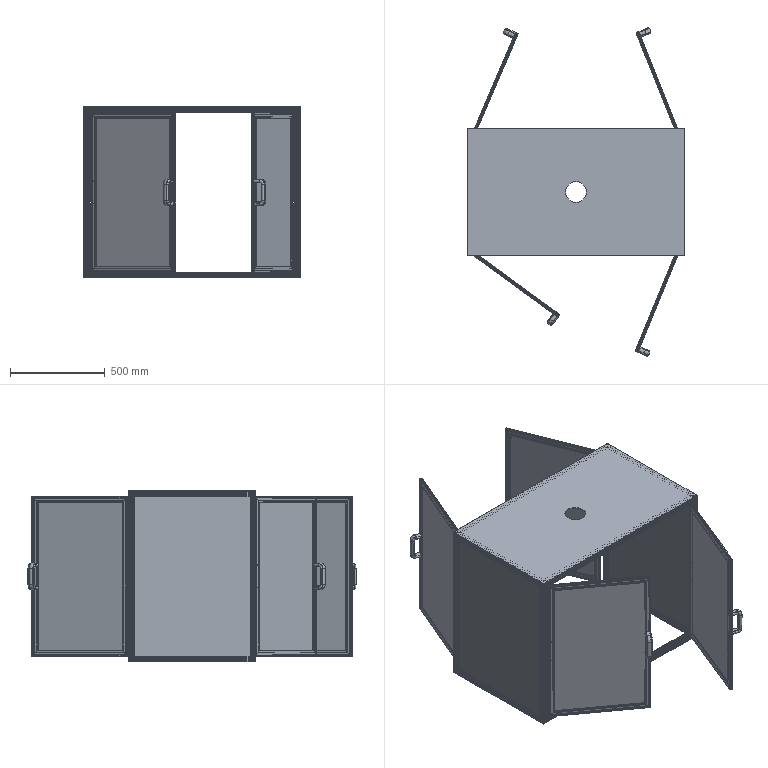Assembly | SolidWorks | mm | 39 component files | 39 solids | 1600 faces | box 1145 x 1728.9 x 905 mm | volume 23832016 mm3 | plane 1146 | cylinder 358 | cone 64 | spline 32 | commonest cylinder face diameters 4.2 x96 0.6 x48 4 x48 5 x32 1 x32 6.8 x24 42 x24 15.54 x20
Bill of materials:
3030-1085 | 4 |  | Long straight prismatic bar with a constant square cross-section: a central round bore, four round corner bores, diagonal webs, and an open slot centered on each of the four faces.
3030-610 | 4 |  | Straight prismatic bar with the same square, four-slot cross-section (central bore, four corner bores, diagonal webs). It looks shorter relative to its section than unnamed part.
3030-900 | 4 |  | Long straight bar with the same square, four-slot cross-section (central bore, four corner bores, diagonal webs), shown standing vertically.
858X628X5 | 2 |  | Thin, flat rectangular plate or sheet with no visible holes or cutouts.
3015-542.5 | 8 |  | Long, narrow slotted strip or profile. Both ends are cut at an angle, giving a trapezoid outline in side view, and grooves run along its length.
3015-840 | 8 |  | Long, slender extrusion with an elongated rectangular cross-section: one central round hole and open lipped slots at both ends and along the sides. The section view appears tilted.
503.5-801-5 | 4 |  | Thin, flat rectangular plate with no visible holes or cutouts.
TopCoverPlate | 1 |  | Thin, flat rectangular plate with one centered circular through-hole.
UPCFN120Handle | 4 |  | U-shaped (bow) handle made of a round-section bar: two parallel legs joined by a straight grip section with rounded bends. Each leg end has a small axial hole.
Mates:
1. coincident | 3030-900-1 face at (1.276, -17.477, 450) dir (0, -1, 0) | 3030-900-2 face at (1097.953, -17.477, 450) dir (0, -1, 0)
2. coincident | 3030-900-1 face at (-27.747, 1.323, 450) dir (0, 0, 1) | 3030-900-2 face at (1087.253, 1.323, 450) dir (0, 0, 1)
3. coincident | 3030-900-1 face at (-27.747, 1.323, 450) dir (0, 0, 1) | 3030-900-4 face at (-27.747, 641.323, 450) dir (0, 0, 1)
4. coincident | 3030-900-1 face at (-28.047, -15.977, 450) dir (-1, 0, 0) | 3030-900-4 face at (-28.047, 641.323, 450) dir (-1, 0, 0)
5. coincident | 3030-900-2 face at (1087.253, 1.323, 450) dir (0, 0, 1) | 3030-900-3 face at (1087.253, 641.323, 450) dir (0, 0, 1)
6. coincident | 3030-900-2 face at (1116.953, -7.277, 450) dir (1, 0, 0) | 3030-900-3 face at (1116.953, 651.023, 450) dir (1, 0, 0)
7. coincident | 3030-900-3 face at (1087.631, 652.523, 450) dir (0, 1, 0) | 3030-900-4 face at (-9.047, 652.523, 450) dir (0, 1, 0)
8. coincident | 3030-900-1 face at (1.953, -7.277, 450) dir (1, 0, 0) | 3030-1085-1 face at (1.953, 1.323, -449.7) dir (-1, 0, 0)
9. coincident | 3030-900-1 face at (1.276, -17.477, 450) dir (0, -1, 0) | 3030-1085-1 face at (1.953, -17.477, -439) dir (0, -1, 0)
10. coincident | 3030-900-1 face at (-27.747, 1.323, -450) dir (0, 0, -1) | 3030-1085-1 face at (1.953, -15.977, -450) dir (0, 0, -1)
11. coincident | 3030-900-2 face at (1086.953, 1.323, 450) dir (-1, 0, 0) | 3030-1085-1 face at (1086.953, 1.323, -449.7) dir (1, 0, 0)
12. coincident | 3030-900-4 face at (1.953, 632.723, 450) dir (1, 0, 0) | 3030-1085-2 face at (1.953, 641.323, -449.7) dir (-1, 0, 0)
13. coincident | 3030-900-4 face at (1.276, 622.523, 450) dir (0, -1, 0) | 3030-1085-2 face at (1.953, 622.523, -439) dir (0, -1, 0)
14. coincident | 3030-900-4 face at (-27.747, 641.323, -450) dir (0, 0, -1) | 3030-1085-2 face at (1.953, 624.023, -450) dir (0, 0, -1)
15. coincident | 3030-900-1 face at (1.953, 11.023, 450) dir (1, 0, 0) | 3030-1085-3 face at (1.953, 1.323, 420.3) dir (-1, 0, 0)
16. coincident | 3030-900-1 face at (1.276, -17.477, 450) dir (0, -1, 0) | 3030-1085-3 face at (1.953, -17.477, 449.323) dir (0, -1, 0)
17. coincident | 3030-900-1 face at (-27.747, 1.323, 450) dir (0, 0, 1) | 3030-1085-3 face at (1.953, 11.023, 450) dir (0, 0, 1)
18. coincident | 3030-900-4 face at (1.953, 632.723, 450) dir (1, 0, 0) | 3030-1085-5 face at (1.953, 641.323, 420.3) dir (-1, 0, 0)
19. coincident | 3030-900-4 face at (1.276, 622.523, 450) dir (0, -1, 0) | 3030-1085-5 face at (1.953, 622.523, 449.323) dir (0, -1, 0)
20. coincident | 3030-900-4 face at (-27.747, 641.323, 450) dir (0, 0, 1) | 3030-1085-5 face at (1.953, 651.023, 450) dir (0, 0, 1)
21. coincident | 3030-1085-2 face at (1.953, 622.523, -439) dir (0, -1, 0) | 3030-610-1 face at (-27.747, 622.523, -438.8) dir (0, 1, 0)
22. coincident | 3030-900-4 face at (-28.047, 624.023, 450) dir (-1, 0, 0) | 3030-610-1 face at (-28.047, 622.523, -438.8) dir (-1, 0, 0)
23. coincident | 3030-900-4 face at (-27.747, 641.323, -450) dir (0, 0, -1) | 3030-610-1 face at (-9.047, 622.523, -450) dir (0, 0, -1)
24. coincident | 3030-900-1 face at (-9.047, 12.523, 450) dir (0, 1, 0) | 3030-610-1 face at (-27.747, 12.523, -438.8) dir (0, -1, 0)
25. coincident | 3030-900-2 face at (1105.953, 12.523, 450) dir (0, 1, 0) | 3030-610-4 face at (1087.253, 12.523, -431.2) dir (0, -1, 0)
26. coincident | 3030-900-2 face at (1116.953, 11.023, 450) dir (1, 0, 0) | 3030-610-4 face at (1116.953, 12.523, -439.8) dir (1, 0, 0)
27. coincident | 3030-900-2 face at (1087.253, 1.323, -450) dir (0, 0, -1) | 3030-610-4 face at (1116.276, 12.523, -450) dir (0, 0, -1)
28. coincident | 3030-900-3 face at (1116.276, 622.523, 450) dir (0, -1, 0) | 3030-610-3 face at (1087.253, 622.523, 431.2) dir (0, 1, 0)
29. coincident | 3030-900-3 face at (1116.953, 651.023, 450) dir (1, 0, 0) | 3030-610-3 face at (1116.953, 622.523, 421.5) dir (1, 0, 0)
30. coincident | 3030-900-3 face at (1087.253, 641.323, 450) dir (0, 0, 1) | 3030-610-3 face at (1097.953, 622.523, 450) dir (0, 0, 1)
31. coincident | 3030-900-4 face at (-17.047, 622.523, 450) dir (0, -1, 0) | 3030-610-2 face at (-27.747, 622.523, 431.2) dir (0, 1, 0)
32. coincident | 3030-900-4 face at (-28.047, 624.023, 450) dir (-1, 0, 0) | 3030-610-2 face at (-28.047, 622.523, 431.2) dir (-1, 0, 0)
33. coincident | 3030-900-4 face at (-27.747, 641.323, 450) dir (0, 0, 1) | 3030-610-2 face at (1.276, 622.523, 450) dir (0, 0, 1)
34. coincident | 3030-610-3 face at (1097.953, 622.523, 450) dir (0, 0, 1) | TopCoverPlate-1 face at (-28.047, 652.523, 450) dir (0, 0, -1)
35. coincident | 3030-610-3 face at (1116.953, 622.523, 439.8) dir (1, 0, 0) | TopCoverPlate-1 face at (1116.953, 652.523, 455) dir (1, 0, 0)
36. coincident | 3030-900-3 face at (1105.953, 652.523, 450) dir (0, 1, 0) | TopCoverPlate-1 face at (-28.047, 652.523, 455) dir (0, 1, 0)
37. coincident | 3030-610-4 face at (1097.368, 12.523, -429) dir (0, 0, 1) | 858X628X5-1 face at (1105.953, 631.523, -429) dir (0, 0, -1)
38. coincident | 3030-900-3 face at (1106.539, 631.523, 450) dir (0, -1, 0) | 858X628X5-1 face at (1105.953, 631.523, 429) dir (0, 1, 0)
39. coincident | 3030-610-4 face at (1105.953, 12.523, -422) dir (-1, 0, 0) | 858X628X5-1 face at (1105.953, 631.523, 429) dir (1, 0, 0)
40. coincident | 3030-610-1 face at (-8.461, 622.523, -429) dir (0, 0, 1) | 858X628X5-2 face at (-17.047, 631.523, -429) dir (0, 0, -1)
41. coincident | 3030-900-1 face at (-17.632, 3.523, 450) dir (0, 1, 0) | 858X628X5-2 face at (-17.047, 3.523, -429) dir (0, -1, 0)
42. coincident | 3030-610-1 face at (-17.047, 622.523, -422) dir (1, 0, 0) | 858X628X5-2 face at (-17.047, 631.523, -429) dir (-1, 0, 0)
43. coincident | 3030-1085-5 face at (1.953, 624.023, 420) dir (0, 0, -1) | GuardDoor-1/3015-542.5-1 face at (1067.141, 655.276, 420) dir (0, 0, 1)
44. coincident | 3030-1085-5 face at (1.953, 624.023, 420) dir (0, 0, -1) | GuardDoor-2/3015-542.5-1 face at (235.292, 1153.537, 420) dir (0, 0, 1)
45. coincident | GuardDoor-1/3015-840-1 face at (875.161, 1162.783, -420) dir (0.9282, 0.3721, 0) | UPCFN120Handle-1 face at (880.742, 1148.86, -60.5) dir (-0.9282, -0.3721, 0)
46. concentric | GuardDoor-1/3015-840-1 face at (867.283, 1143.465, 60) dir (-0.9282, -0.3721, 0) r 0.5 | UPCFN120Handle-1 face at (891.874, 1153.323, 60) dir (-0.9282, -0.3721, 0) r 3.324
47. concentric | GuardDoor-1/3015-840-1 face at (867.283, 1143.465, -60) dir (-0.9282, -0.3721, 0) r 0.5 | UPCFN120Handle-1 face at (891.874, 1153.323, -60) dir (-0.9282, -0.3721, 0) r 3.324
48. coincident | GuardDoor-2/3015-840-2 face at (225.502, 1157.731, -420) dir (-0.9192, 0.3938, 0) | UPCFN120Handle-2 face at (219.596, 1143.943, -60.5) dir (0.9192, -0.3938, 0)
49. concentric | GuardDoor-2/3015-840-2 face at (220.055, 1143.746, -60) dir (-0.9192, 0.3938, 0) r 0.5 | UPCFN120Handle-2 face at (208.572, 1148.666, -60) dir (0.9192, -0.3938, 0) r 3.324
50. concentric | GuardDoor-2/3015-840-2 face at (220.055, 1143.746, 60) dir (-0.9192, 0.3938, 0) r 0.5 | UPCFN120Handle-2 face at (208.572, 1148.666, 60) dir (0.9192, -0.3938, 0) r 3.324
51. coincident | 3030-1085-3 face at (1.953, 1.323, 420) dir (0, 0, -1) | GuardDoor-4/3015-542.5-1 face at (457.672, -327.96, 420) dir (0, 0, 1)
52. coincident | 3030-1085-3 face at (1.953, -15.977, 420) dir (0, 0, -1) | GuardDoor-3/3015-542.5-1 face at (1063.157, -18.418, 420) dir (0, 0, 1)
53. coincident | GuardDoor-3/3015-840-1 face at (870.61, -525.82, -420) dir (0.9248, -0.3805, 0) | UPCFN120Handle-3 face at (876.318, -511.948, -60.5) dir (-0.9248, 0.3805, 0)
54. concentric | GuardDoor-3/3015-840-1 face at (875.855, -511.758, 60) dir (0.9248, -0.3805, 0) r 0.5 | UPCFN120Handle-3 face at (887.409, -516.512, 60) dir (-0.9248, 0.3805, 0) r 3.324
55. concentric | GuardDoor-3/3015-840-1 face at (875.855, -511.758, -60) dir (0.9248, -0.3805, 0) r 0.5 | UPCFN120Handle-3 face at (887.409, -516.512, -60) dir (-0.9248, 0.3805, 0) r 3.324
56. coincident | GuardDoor-4/3015-840-2 face at (448.83, -340.077, -420) dir (-0.5895, -0.8078, 0) | UPCFN120Handle-4 face at (436.713, -331.236, 60.5) dir (0.5895, 0.8078, 0)
57. concentric | GuardDoor-4/3015-840-2 face at (445.26, -319.522, 60) dir (0.5895, 0.8078, 0) r 0.5 | UPCFN120Handle-4 face at (429.643, -340.923, 60) dir (0.5895, 0.8078, 0) r 3.324
58. concentric | GuardDoor-4/3015-840-2 face at (445.26, -319.522, -60) dir (0.5895, 0.8078, 0) r 0.5 | UPCFN120Handle-4 face at (429.643, -340.923, -60) dir (0.5895, 0.8078, 0) r 3.324
59. coincident | 3030-1085-5 face at (1.953, 624.023, 420) dir (0, 0, -1) | GuardDoor-1/3015-542.5-1 face at (1077.026, 659.239, 420) dir (0, 0, 1)
60. coincident | 3015-542.5-1 face at (-16.364, -10.026, -271.25) dir (0.7071, 0, -0.7071) | 3015-840-1 face at (13.636, 29.974, -241.25) dir (-0.7071, 0, 0.7071)
61. coincident | 3015-542.5-1 face at (-16.364, 7.974, 271.25) dir (0, 1, 0) | 3015-840-1 face at (823.636, 7.974, -271.25) dir (0, 1, 0)
62. coincident | 3015-542.5-1 face at (-16.364, 7.974, 271.25) dir (-1, 0, 0) | 3015-840-1 edge at (-16.364, 3.624, -271.25) dir (0, 1, 0)
63. coincident | 3015-542.5-1 face at (-16.364, 7.974, 271.25) dir (0, 1, 0) | 3015-840-2 face at (823.636, 7.974, 271.25) dir (0, 1, 0)
64. coincident | 3015-542.5-1 face at (-16.364, -10.026, 271.25) dir (0.7071, 0, 0.7071) | 3015-840-2 face at (13.636, -29.026, 241.25) dir (-0.7071, 0, -0.7071)
65. coincident | 3015-542.5-1 face at (-16.364, 7.974, 271.25) dir (-1, 0, 0) | 3015-840-2 edge at (-16.364, 7.974, 271.25) dir (0, -1, 0)
66. coincident | 3015-840-2 face at (823.636, -7.026, 271.25) dir (0, -1, 0) | 3015-542.5-2 face at (823.636, -7.026, 271.25) dir (0, -1, 0)
67. coincident | 3015-840-2 face at (823.636, -13.026, 271.25) dir (0.7071, 0, -0.7071) | 3015-542.5-2 face at (823.636, 10.974, 271.25) dir (-0.7071, 0, 0.7071)
68. coincident | 3015-840-2 face at (823.636, 7.974, 271.25) dir (0, 0, 1) | 3015-542.5-2 edge at (823.636, 3.624, 271.25) dir (0, 1, 0)
69. coincident | 3015-542.5-1 face at (3.136, 3.624, 271.25) dir (1, 0, 0) | 503.5-801-5-1 face at (3.136, 3.624, 251.75) dir (-1, 0, 0)
70. coincident | 3015-840-2 face at (823.636, 3.624, 251.75) dir (0, 0, -1) | 503.5-801-5-1 face at (3.136, 3.624, 251.75) dir (0, 0, 1)
71. coincident | 3015-542.5-1 face at (13.636, 3.624, 271.25) dir (0, -1, 0) | 503.5-801-5-1 face at (3.136, 3.624, 251.75) dir (0, 1, 0)